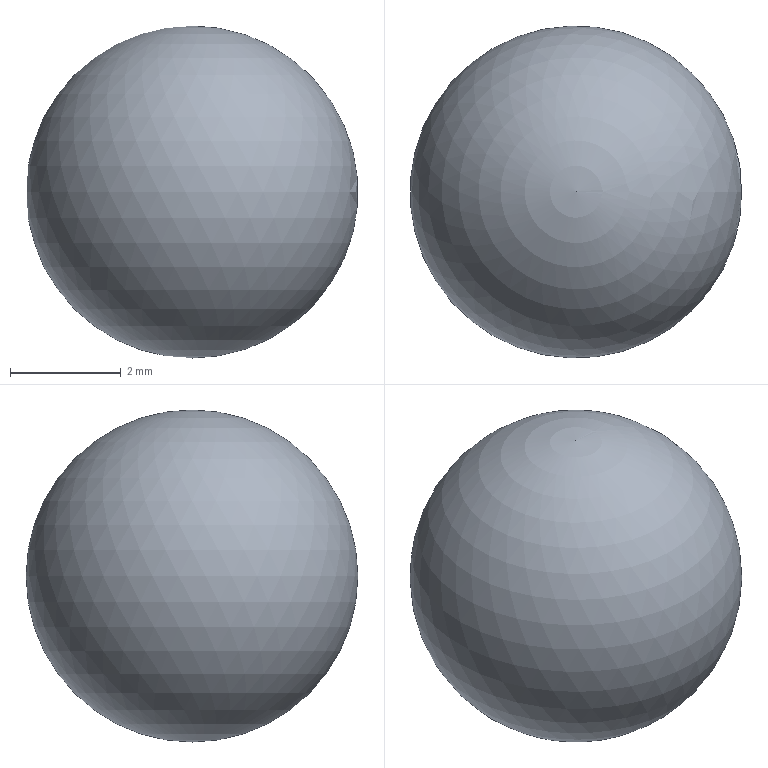Component | NX | BALL_6 | 1 solid | 1 faces | box 6 x 6 x 6 mm | volume 113 mm3 | sphere 1
STEP:
#1=CARTESIAN_POINT('',(0.,0.,0.));
#2=DIRECTION('',(0.,0.,1.));
#3=DIRECTION('',(1.,0.,0.));
#4=AXIS2_PLACEMENT_3D('',#1,#2,#3);
#5=CARTESIAN_POINT('',(0.,-0.,26.031));
#6=VERTEX_POINT('',#5);
#7=VERTEX_LOOP('',#6);
#8=FACE_BOUND('',#7,.T.);
#9=CARTESIAN_POINT('',(0.,-0.,29.031));
#10=DIRECTION('',(0.,0.,1.));
#11=DIRECTION('',(1.,0.,-0.));
#12=AXIS2_PLACEMENT_3D('',#9,#10,#11);
#13=SPHERICAL_SURFACE('',#12,3.);
#14=ADVANCED_FACE('',(#8),#13,.T.);
#15=CLOSED_SHELL('',(#14));
#16=MANIFOLD_SOLID_BREP('',#15);
#17=(LENGTH_UNIT()NAMED_UNIT(*)SI_UNIT(.MILLI.,.METRE.));
#18=UNCERTAINTY_MEASURE_WITH_UNIT(LENGTH_MEASURE(0.0000001),#17,'','');
#19=(NAMED_UNIT(*)PLANE_ANGLE_UNIT()SI_UNIT($,.RADIAN.));
#20=(NAMED_UNIT(*)SI_UNIT($,.STERADIAN.)SOLID_ANGLE_UNIT());
#21=(GEOMETRIC_REPRESENTATION_CONTEXT(3)GLOBAL_UNCERTAINTY_ASSIGNED_CONTEXT((#18))GLOBAL_UNIT_ASSIGNED_CONTEXT((#17,#19,#20))REPRESENTATION_CONTEXT('',''));
#22=ADVANCED_BREP_SHAPE_REPRESENTATION('',(#4,#16),#21);